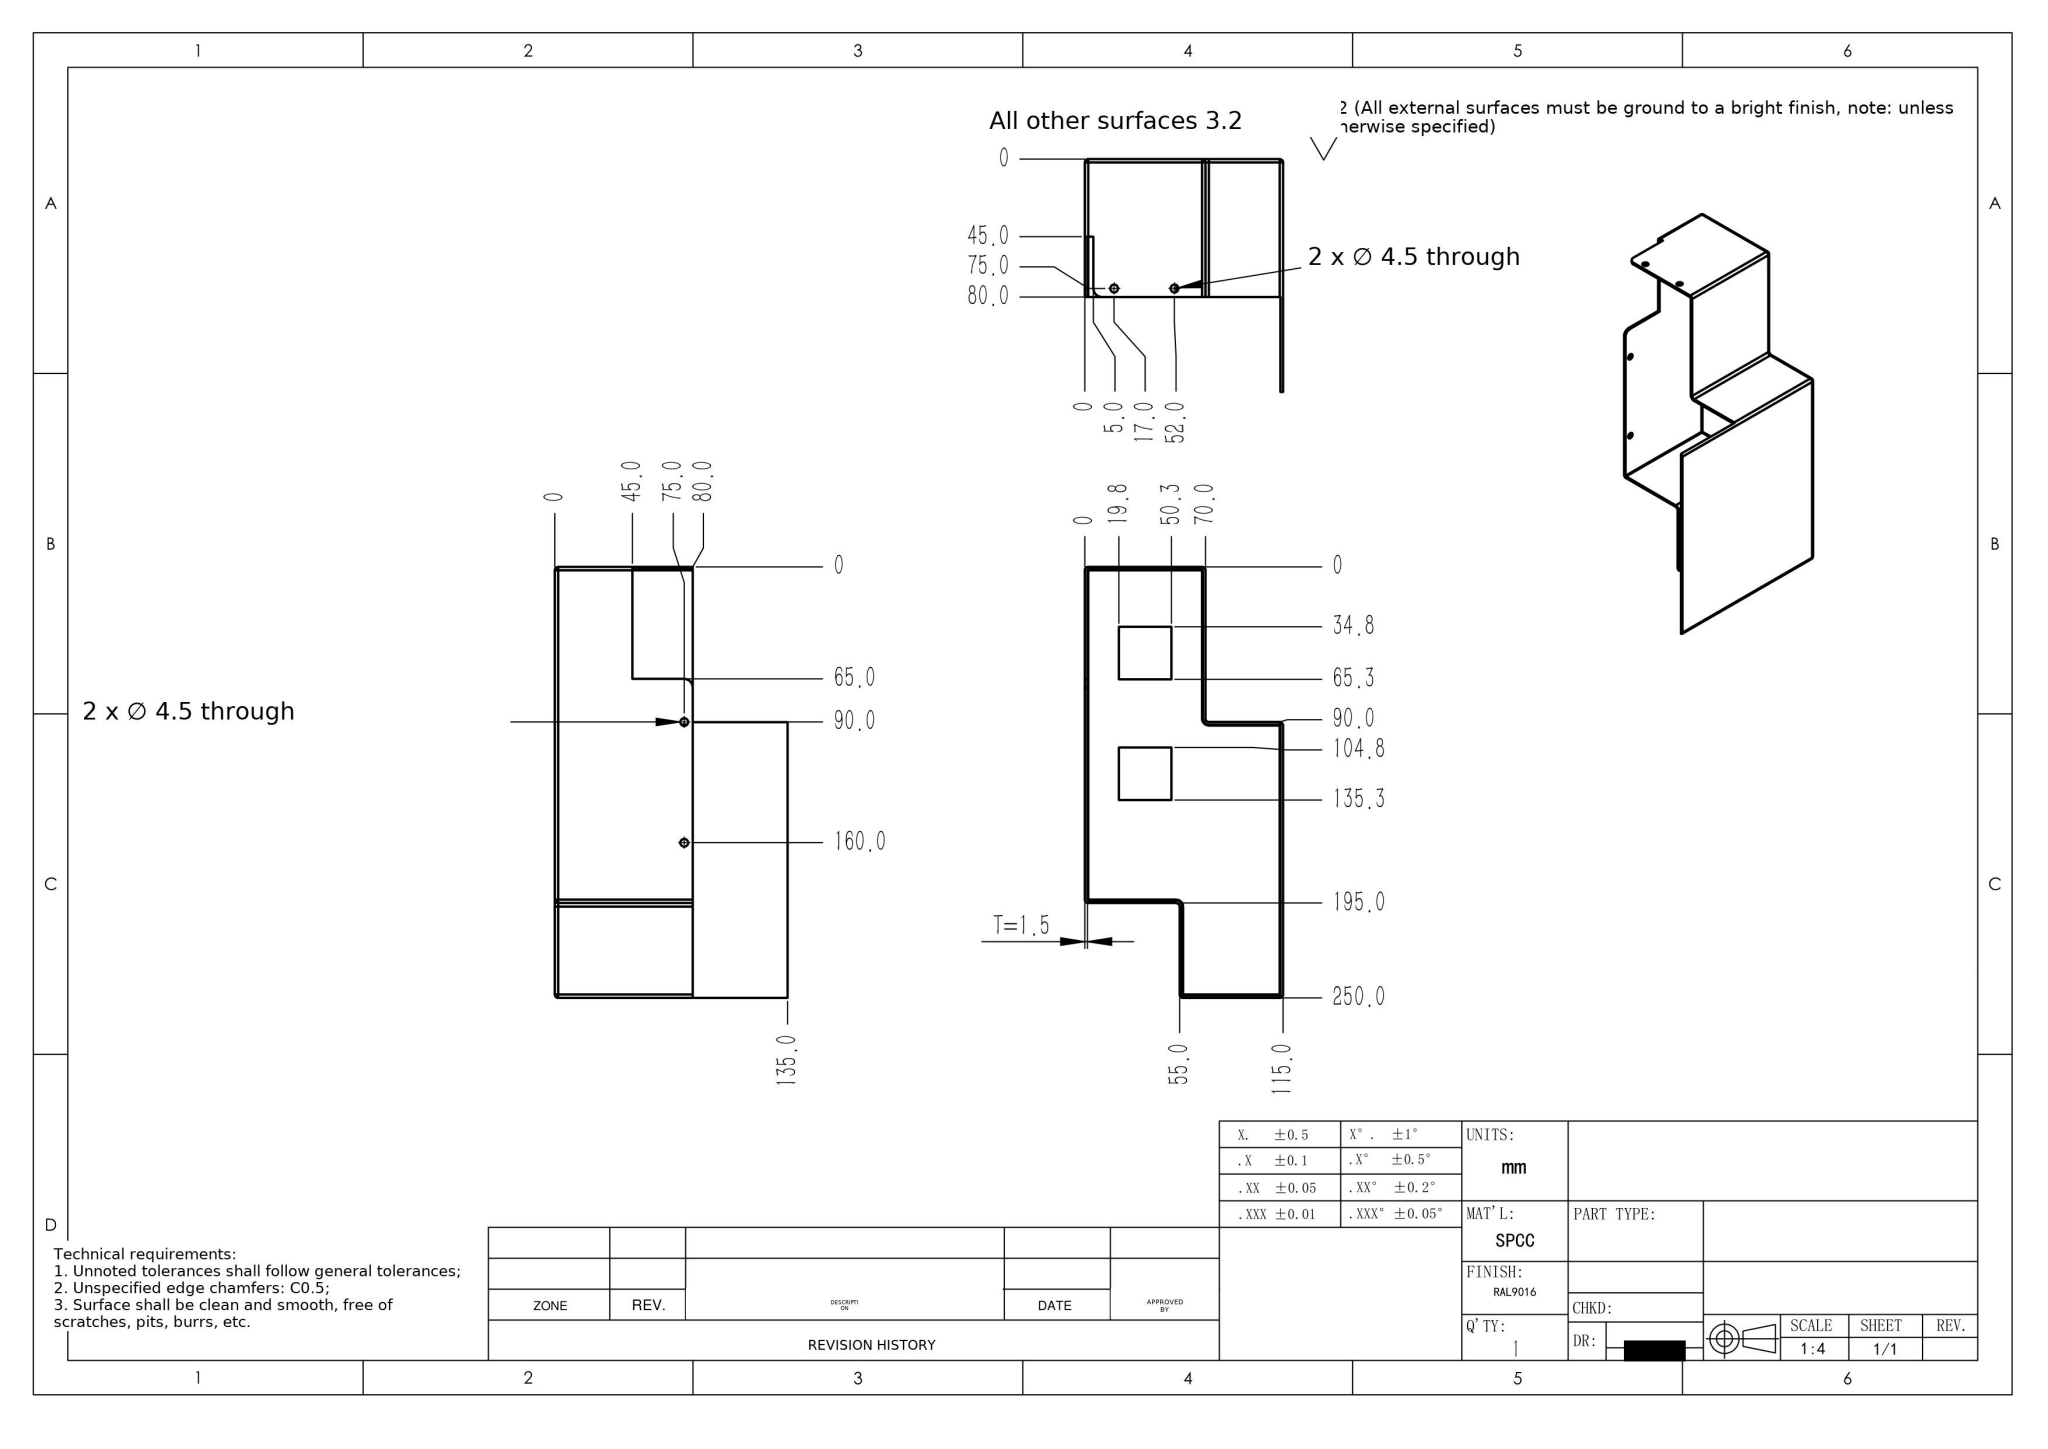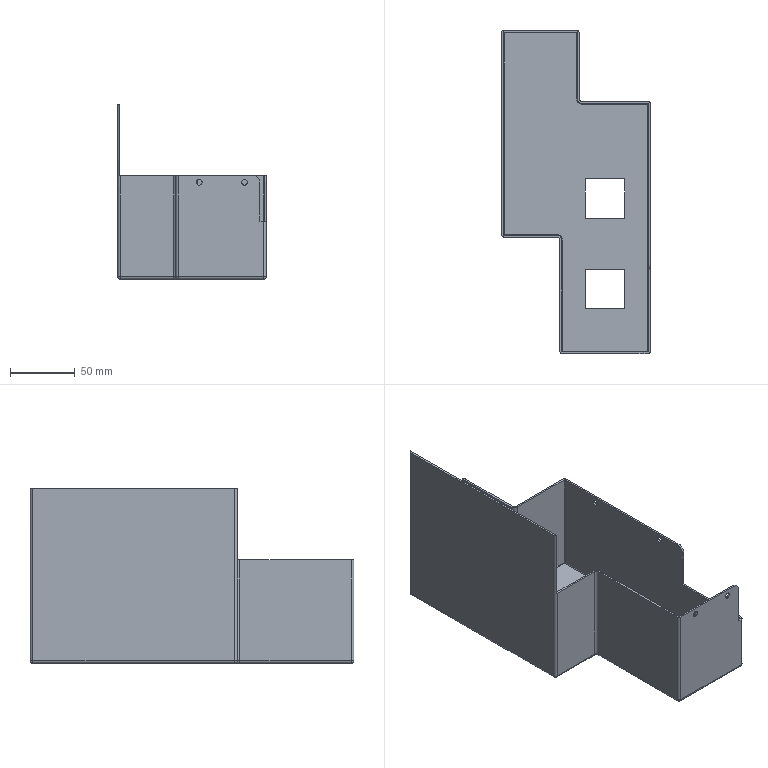Part | SolidWorks | mm | material SPCC | 1 solid | 91 faces | box 115 x 250 x 135 mm | volume 119734 mm3 | cylinder 42 | plane 33 | sphere 12 | torus 4 | commonest cylinder face diameters 4 x16 1 x14 4.5 x8 7 x2 10 x2
build123d program:
from build123d import *

# Parameters (mm, degrees)
SKETCH1_W                = 115
SKETCH1_H                = 250
BOSS_EXTRUDE1_DEPTH      = 135
SKETCH4_W                = 45
SKETCH4_H                = 90
SKETCH4_W_2              = 55
SKETCH4_H_2              = 55
CUT_EXTRUDE3_DEPTH       = 290.881
FILLET1_R                = 2
SHELL1_T                 = -1.5
SKETCH2_W                = 57
SKETCH2_H                = 5
CUT_EXTRUDE1_DEPTH       = 95
SKETCH3_W                = 113.5
SKETCH3_H                = 250
CUT_EXTRUDE2_DEPTH       = 55
SKETCH5_W                = 35
SKETCH5_H                = 65
CUT_EXTRUDE4_DEPTH       = 5
M4_CLEARANCE_HOLE1_D     = 4.5
M4_CLEARANCE_HOLE1_DEPTH = 1.5
M4_CLEARANCE_HOLE2_D     = 4.5
M4_CLEARANCE_HOLE2_DEPTH = 1.5
CUT_EXTRUDE5_REACH       = 291.881
SKETCH10_W               = 30.5
SKETCH10_H               = 30.5
FILLET2_R                = 5


with BuildPart() as part:
    # Sketch1 → Boss-Extrude1 (new body)
    with BuildSketch(Plane.XY):
        with Locations((0, 125)):
            Rectangle(SKETCH1_W, SKETCH1_H)
    extrude(amount=BOSS_EXTRUDE1_DEPTH)

    # Sketch4 → Cut-Extrude3 (cut, through all)
    with BuildSketch(Plane(origin=(0, 0, 0), x_dir=(-1, 0, 0), z_dir=(0, 0, -1))):
        with Locations((35, 45)):
            Rectangle(SKETCH4_W, SKETCH4_H)
        with Locations((-30, 222.5)):
            Rectangle(SKETCH4_W_2, SKETCH4_H_2)
    extrude(amount=-CUT_EXTRUDE3_DEPTH, mode=Mode.SUBTRACT)

    # Fillet1
    fillet1_edges = [part.edges().sort_by_distance(p)[0] for p in [
        (22.5, 0, 0),
        (-57.5, 90, 67.5),
        (-12.5, 0, 67.5),
        (-12.5, 90, 67.5),
        (-35, 90, 0),
        (-12.5, 45, 0),
        (-27.5, 250, 0),
        (57.5, 195, 67.5),
        (2.5, 250, 67.5),
        (2.5, 195, 67.5),
        (30, 195, 0),
        (2.5, 222.5, 0),
        (57.5, 97.5, 0),
        (-57.5, 170, 0),
        (-57.5, 250, 67.5),
        (57.5, 0, 67.5),
    ]]
    fillet(fillet1_edges, radius=FILLET1_R)

    # Shell1
    shell1_openings = [part.faces().sort_by_distance(p)[0] for p in [
        (2.353, 126.341, 135),
    ]]
    offset(amount=SHELL1_T, openings=shell1_openings, kind=Kind.INTERSECTION)

    # Sketch2 → Cut-Extrude1 (cut)
    with BuildSketch(Plane.XY.offset(135)):
        with Locations((-27.5, 247.5)):
            Rectangle(SKETCH2_W, SKETCH2_H)
    extrude(amount=-CUT_EXTRUDE1_DEPTH, mode=Mode.SUBTRACT)

    # Sketch3 → Cut-Extrude2 (cut)
    with BuildSketch(Plane.XY.offset(135)):
        with Locations((0.75, 125)):
            Rectangle(SKETCH3_W, SKETCH3_H)
    extrude(amount=-CUT_EXTRUDE2_DEPTH, mode=Mode.SUBTRACT)

    # Sketch5 → Cut-Extrude4 (cut)
    with BuildSketch(Plane(origin=(57.5, 0, 0), x_dir=(0, 0, -1), z_dir=(1, 0, 0))):
        with Locations((-62.5, 32.5)):
            Rectangle(SKETCH5_W, SKETCH5_H)
    extrude(amount=-CUT_EXTRUDE4_DEPTH, mode=Mode.SUBTRACT)

    # M4 Clearance Hole1
    with Locations(Plane(origin=(0, 0, 0), x_dir=(-1, 0, 0), z_dir=(0, -1, 0))):
        with Locations((-5.5, -75), (-40.5, -75)):
            Hole(M4_CLEARANCE_HOLE1_D / 2, depth=M4_CLEARANCE_HOLE1_DEPTH)

    # M4 Clearance Hole2
    with Locations(Plane(origin=(57.5, 0, 0), x_dir=(0, 0, -1), z_dir=(1, 0, 0))):
        with Locations((-75, 90), (-75, 160)):
            Hole(M4_CLEARANCE_HOLE2_D / 2, depth=M4_CLEARANCE_HOLE2_DEPTH)

    # Sketch10 → Cut-Extrude5 (cut, up to next)
    with BuildSketch(Plane(origin=(0, 0, 0), x_dir=(-1, 0, 0), z_dir=(0, 0, -1)), mode=Mode.PRIVATE) as cut_extrude5_sk1:
        with Locations((-22.5, 50)):
            Rectangle(SKETCH10_W, SKETCH10_H)
    cut_extrude5_tool1 = extrude(cut_extrude5_sk1.sketch, amount=-CUT_EXTRUDE5_REACH, mode=Mode.PRIVATE) & part.part
    # Sketch10 → Cut-Extrude5 (cut, up to next)
    with BuildSketch(Plane(origin=(0, 0, 0), x_dir=(-1, 0, 0), z_dir=(0, 0, -1)), mode=Mode.PRIVATE) as cut_extrude5_sk2:
        with Locations((-22.5, 120)):
            Rectangle(SKETCH10_W, SKETCH10_H)
    cut_extrude5_tool2 = extrude(cut_extrude5_sk2.sketch, amount=-CUT_EXTRUDE5_REACH, mode=Mode.PRIVATE) & part.part
    add(cut_extrude5_tool1.solids().sort_by_distance((22.5, 50, 0))[0], mode=Mode.SUBTRACT)
    add(cut_extrude5_tool2.solids().sort_by_distance((22.5, 120, 0))[0], mode=Mode.SUBTRACT)

    # Fillet2
    fillet2_edges = [part.edges().sort_by_distance(p)[0] for p in [
        (52.5, 0.75, 80),
        (56.75, 65, 80),
    ]]
    fillet(fillet2_edges, radius=FILLET2_R)


solid = part.part